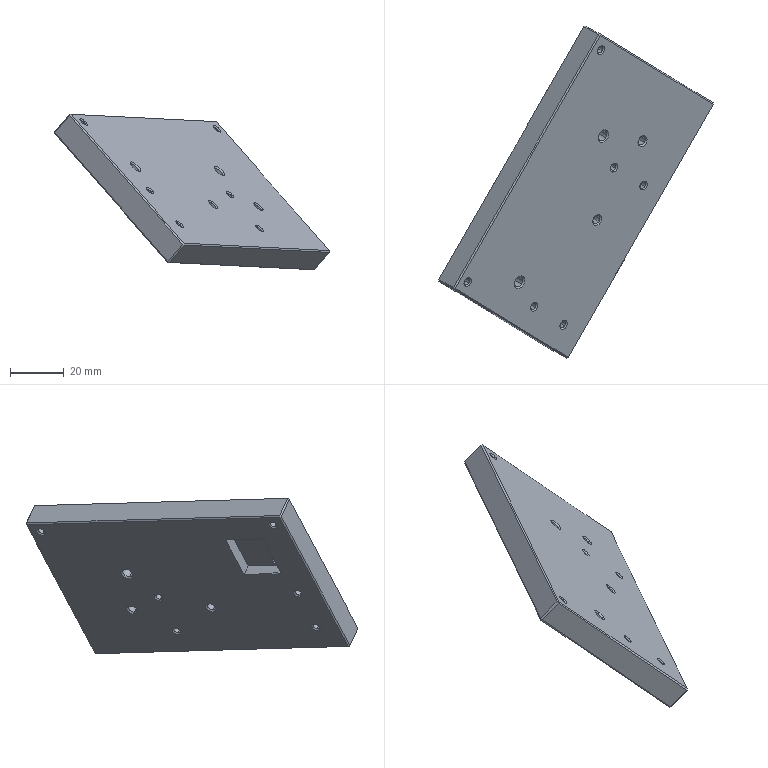Component | SolidWorks | 7z0-123-1 | 1 solid | 107 faces | box 102.62 x 123.99 x 58.08 mm | volume 74449 mm3 | cone 48 | plane 31 | cylinder 28 | commonest cylinder face diameters 2.5 x12 3.3 x8 4 x8
build123d program:
from build123d import *

# Parameters (mm, degrees)
SKETCH1_2_W                   = 70
SKETCH1_2_H                   = 110
BOSS_EXTRUDE1_DEPTH           = 10
M4_TAPPED_HOLE1_D             = 3.3
M4_TAPPED_HOLE1_DEPTH         = 10.1
M4_TAPPED_HOLE1_TIP           = 0.9914
SIZE_MM_DOWEL_PIN_HOLE1_D     = 4
SIZE_MM_DOWEL_PIN_HOLE1_DEPTH = 10
SIZE_MM_DOWEL_PIN_HOLE1_TIP   = 1.202
M3_TAPPED_HOLE1_D             = 2.5
SIZE_MM_DOWEL_PIN_HOLE2_D     = 4
SIZE_MM_DOWEL_PIN_HOLE2_DEPTH = 10
SIZE_MM_DOWEL_PIN_HOLE2_TIP   = 1.202
M4_TAPPED_HOLE2_D             = 3.3
M3_TAPPED_HOLE2_D             = 2.5
CHAMFER1_SIZE                 = 0.5
SKETCH1_W                     = 18.5
SKETCH1_H                     = 16
FLAGRELIEFPOCKET_DEPTH        = 4.5


with BuildPart() as part:
    # Sketch1_2 → Boss-Extrude1 (new body)
    with BuildSketch(Plane.XY):
        Rectangle(SKETCH1_2_W, SKETCH1_2_H)
    extrude(amount=BOSS_EXTRUDE1_DEPTH)

    # M4 Tapped Hole1
    with Locations(Plane(origin=(0, -55, 0), x_dir=(-1, 0, 0), z_dir=(0, -1, 0))):
        with Locations((-27, -5), (3, -5)):
            Hole(M4_TAPPED_HOLE1_D / 2, depth=M4_TAPPED_HOLE1_DEPTH)
            with Locations((0, 0, -(M4_TAPPED_HOLE1_DEPTH + M4_TAPPED_HOLE1_TIP / 2))):  # 118° drill point
                Cone(0, M4_TAPPED_HOLE1_D / 2, M4_TAPPED_HOLE1_TIP, mode=Mode.SUBTRACT)

    # Size mm Dowel Pin Hole1
    with Locations(Plane(origin=(0, -55, 0), x_dir=(-1, 0, 0), z_dir=(0, -1, 0))):
        with Locations((-17, -5), (-7, -5)):
            Hole(SIZE_MM_DOWEL_PIN_HOLE1_D / 2, depth=SIZE_MM_DOWEL_PIN_HOLE1_DEPTH)
            with Locations((0, 0, -(SIZE_MM_DOWEL_PIN_HOLE1_DEPTH + SIZE_MM_DOWEL_PIN_HOLE1_TIP / 2))):  # 118° drill point
                Cone(0, SIZE_MM_DOWEL_PIN_HOLE1_D / 2, SIZE_MM_DOWEL_PIN_HOLE1_TIP, mode=Mode.SUBTRACT)

    # M3 Tapped Hole1 (through all)
    with Locations(Plane.XY.offset(10)):
        with Locations((24, -15), (6, 45), (24, 45), (6, -15)):
            Hole(M3_TAPPED_HOLE1_D / 2)

    # Size mm Dowel Pin Hole2
    with Locations(Plane.XY.offset(10)):
        with Locations((-7, -23), (-7, 40)):
            Hole(SIZE_MM_DOWEL_PIN_HOLE2_D / 2, depth=SIZE_MM_DOWEL_PIN_HOLE2_DEPTH)
            with Locations((0, 0, -(SIZE_MM_DOWEL_PIN_HOLE2_DEPTH + SIZE_MM_DOWEL_PIN_HOLE2_TIP / 2))):  # 118° drill point
                Cone(0, SIZE_MM_DOWEL_PIN_HOLE2_D / 2, SIZE_MM_DOWEL_PIN_HOLE2_TIP, mode=Mode.SUBTRACT)

    # M4 Tapped Hole2 (through all)
    with Locations(Plane(origin=(0, 0, 0), x_dir=(-1, 0, 0), z_dir=(0, 0, -1))):
        with Locations((-12, -29), (-12, 5)):
            Hole(M4_TAPPED_HOLE2_D / 2)

    # M3 Tapped Hole2 (through all)
    with Locations(Plane(origin=(0, 0, 0), x_dir=(-1, 0, 0), z_dir=(0, 0, -1))):
        with Locations((30.5, 50), (30.5, -50)):
            Hole(M3_TAPPED_HOLE2_D / 2)

    # Chamfer1
    chamfer1_edges = [part.edges().sort_by_distance(p)[0] for p in [
        (-35, 0, 10),
        (0, -55, 10),
        (7.25, -15, 10),
        (7.25, -15, 0),
        (35, 0, 10),
        (25.25, 45, 10),
        (25.25, 45, 0),
        (0, -55, 0),
        (7.25, 45, 10),
        (7.25, 45, 0),
        (-35, 0, 0),
        (25.25, -15, 10),
        (25.25, -15, 0),
        (0, 55, 0),
        (-5, 40, 10),
        (-5, 40, 0),
        (35, 0, 0),
        (-5, -23, 10),
        (-5, -23, 0),
        (10.35, 5, 0),
        (10.35, 5, 10),
        (0, 55, 10),
        (10.35, -29, 0),
        (10.35, -29, 10),
        (35, -55, 5),
        (-35, -55, 5),
        (-35, 55, 5),
        (35, 55, 5),
        (-31.75, -50, 0),
        (-31.75, -50, 10),
        (-31.75, 50, 0),
        (-31.75, 50, 10),
    ]]
    chamfer(chamfer1_edges, length=CHAMFER1_SIZE)

    # Sketch1 → FlagReliefPocket (cut)
    with BuildSketch(Plane.XY.offset(10)):
        with Locations((-14.25, 34.5)):
            Rectangle(SKETCH1_W, SKETCH1_H)
    extrude(amount=-FLAGRELIEFPOCKET_DEPTH, mode=Mode.SUBTRACT)


solid = part.part

# Placed as in the assembly
solid = solid.moved(Location((-0.1369, -82.082, 163.051), (-155.101, -37.93, 39.124)))